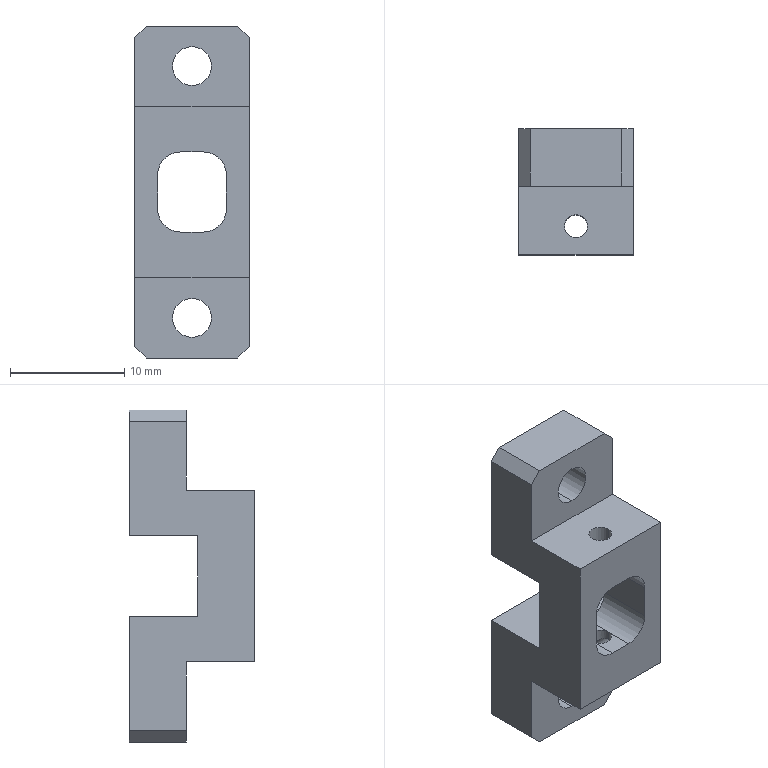Component | SolidWorks | SAWH02-03111A0TensionSpringMountingBlock-1 | 1 solid | 39 faces | box 10 x 11 x 29 mm | volume 1590 mm3 | plane 25 | cylinder 14 | commonest cylinder face diameters 2 x4 3.4 x4 4 x4 2.5 x2 | material Q235A